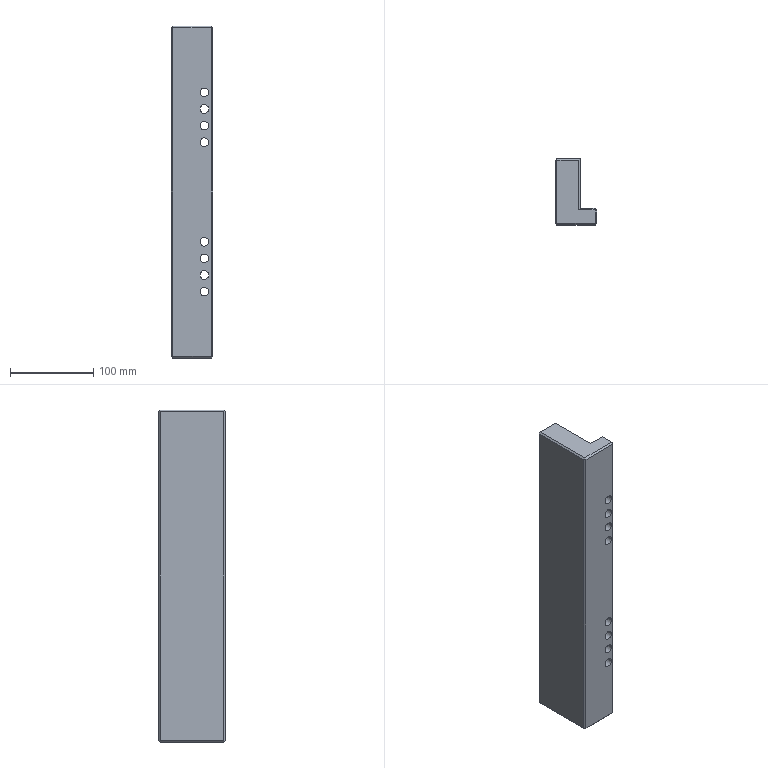Component | SolidWorks | DieShim-1 | 1 solid | 80 faces | box 50 x 80 x 400 mm | volume 1088749 mm3 | cylinder 34 | plane 28 | cone 18 | commonest cylinder face diameters 8.5 x18 10.5 x16
build123d program:
from build123d import *

# Parameters (mm, degrees)
BOSS_EXTRUDE1_DEPTH = 400
LPATTERN1_COUNT     = 5
LPATTERN1_PITCH     = 40
LPATTERN2_COUNT     = 5
LPATTERN2_PITCH     = 40
SKETCH4_R           = 5.25
CUT_EXTRUDE1_DEPTH  = 408.554
CHAMFER1_SIZE       = 2
CHAMFER2_SIZE       = 2


with BuildPart() as part:
    # Sketch1 → Boss-Extrude1 (new body)
    with BuildSketch(Plane.XY):
        Polygon((0, 0), (-80, 0), (-80, -30), (-20, -30), (-20, -50), (0, -50), (0, -21.326), align=None)
    extrude(amount=BOSS_EXTRUDE1_DEPTH)

    # Sketch2 → M10 Tapped Hole1 (revolve, cut)
    with BuildSketch(Plane(origin=(-80, -15, 200), x_dir=(0, 0, 1), z_dir=(0, 1, 0))):
        Polygon((0, 0), (0, 27.554), (4.25, 25), (4.25, 0), align=None)
    m10_tapped_hole1 = revolve(axis=Axis((-86.35, -15, 200), (1, 0, 0)), mode=Mode.SUBTRACT)

    # LPattern1: M10 Tapped Hole1 ×5
    with Locations(*[(0, 0, -i * LPATTERN1_PITCH) for i in range(1, LPATTERN1_COUNT)]):
        add(m10_tapped_hole1, mode=Mode.SUBTRACT)

    # LPattern2: M10 Tapped Hole1 ×5
    with Locations(*[(0, 0, i * LPATTERN2_PITCH) for i in range(1, LPATTERN2_COUNT)]):
        add(m10_tapped_hole1, mode=Mode.SUBTRACT)

    # Sketch4 → Cut-Extrude1 (cut, through all)
    with BuildSketch(Plane.ZY.offset(20)):
        with Locations(Location((140, -40, 0), (0, 0, 270))):
            Circle(SKETCH4_R)
        with Locations(Location((120, -40, 0), (0, 0, 270))):
            Circle(SKETCH4_R)
        with Locations(Location((100, -40, 0), (0, 0, 270))):
            Circle(SKETCH4_R)
        with Locations(Location((80, -40, 0), (0, 0, 270))):
            Circle(SKETCH4_R)
        with Locations(Location((320, -40, 0), (0, 0, 90))):
            Circle(SKETCH4_R)
        with Locations(Location((300, -40, 0), (0, 0, 90))):
            Circle(SKETCH4_R)
        with Locations(Location((280, -40, 0), (0, 0, 90))):
            Circle(SKETCH4_R)
        with Locations(Location((260, -40, 0), (0, 0, 90))):
            Circle(SKETCH4_R)
    extrude(amount=-CUT_EXTRUDE1_DEPTH, mode=Mode.SUBTRACT)

    # Chamfer1
    chamfer1_edges = [part.edges().sort_by_distance(p)[0] for p in [
        (-80, -15, 400),
        (0, -50, 200),
        (-20, -50, 200),
        (-50, -30, 400),
        (-20, -40, 400),
        (-10, -50, 400),
        (0, -25, 400),
        (0, -25, 0),
        (-40, 0, 400),
        (-10, -50, 0),
        (-20, -40, 0),
        (-50, -30, 0),
        (-80, -15, 0),
        (-40, 0, 0),
    ]]
    chamfer(chamfer1_edges, length=CHAMFER1_SIZE)

    # Chamfer2
    chamfer2_edges = [part.edges().sort_by_distance(p)[0] for p in [
        (-80, 0, 200),
        (0, 0, 200),
    ]]
    chamfer(chamfer2_edges, length=CHAMFER2_SIZE)


solid = part.part

# Placed as in the assembly
solid = solid.moved(Location((-77.951, 317.323, 205), (180, 0, 90)))